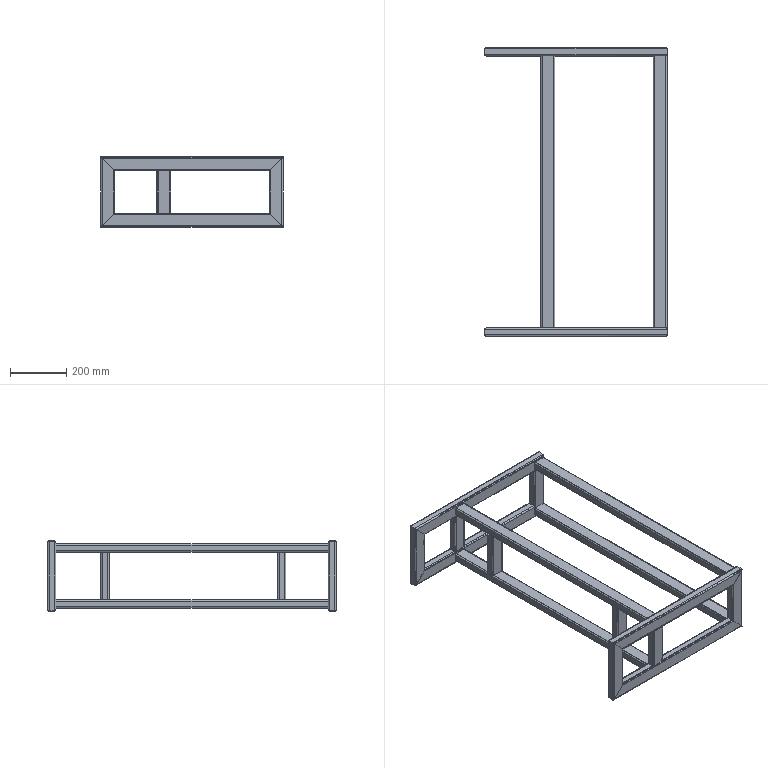Component | SolidWorks | FlipMechanismFixingBracket-1 | 16 solids | 288 faces | volume 2868378 mm3 | plane 160 | cylinder 128 | commonest cylinder face diameters 10.4 x64 5.2 x64